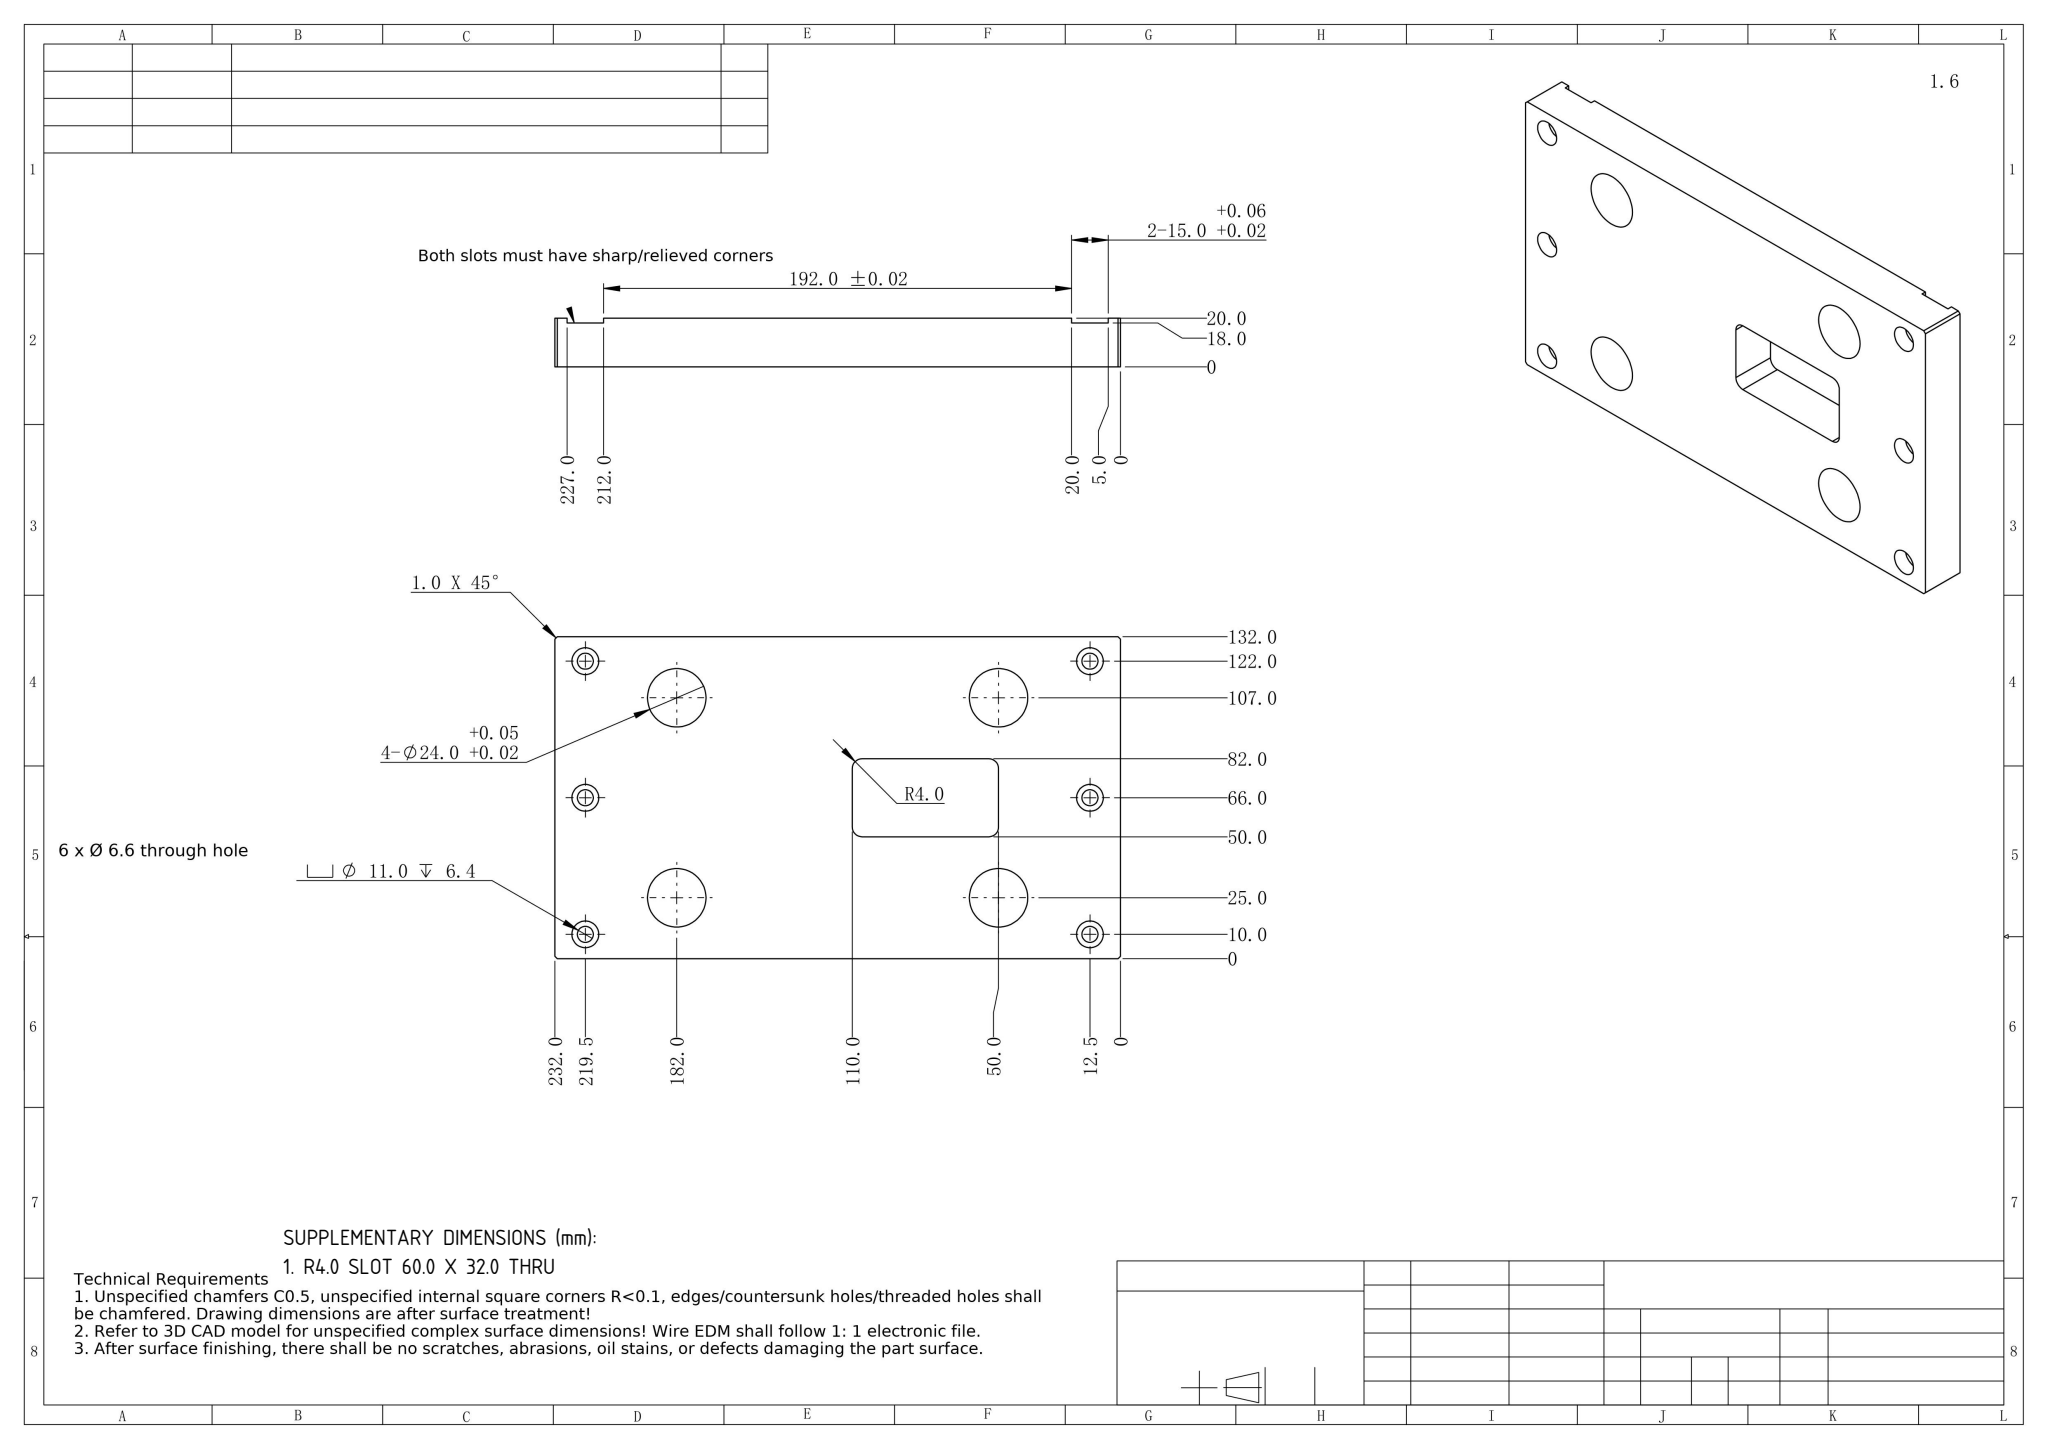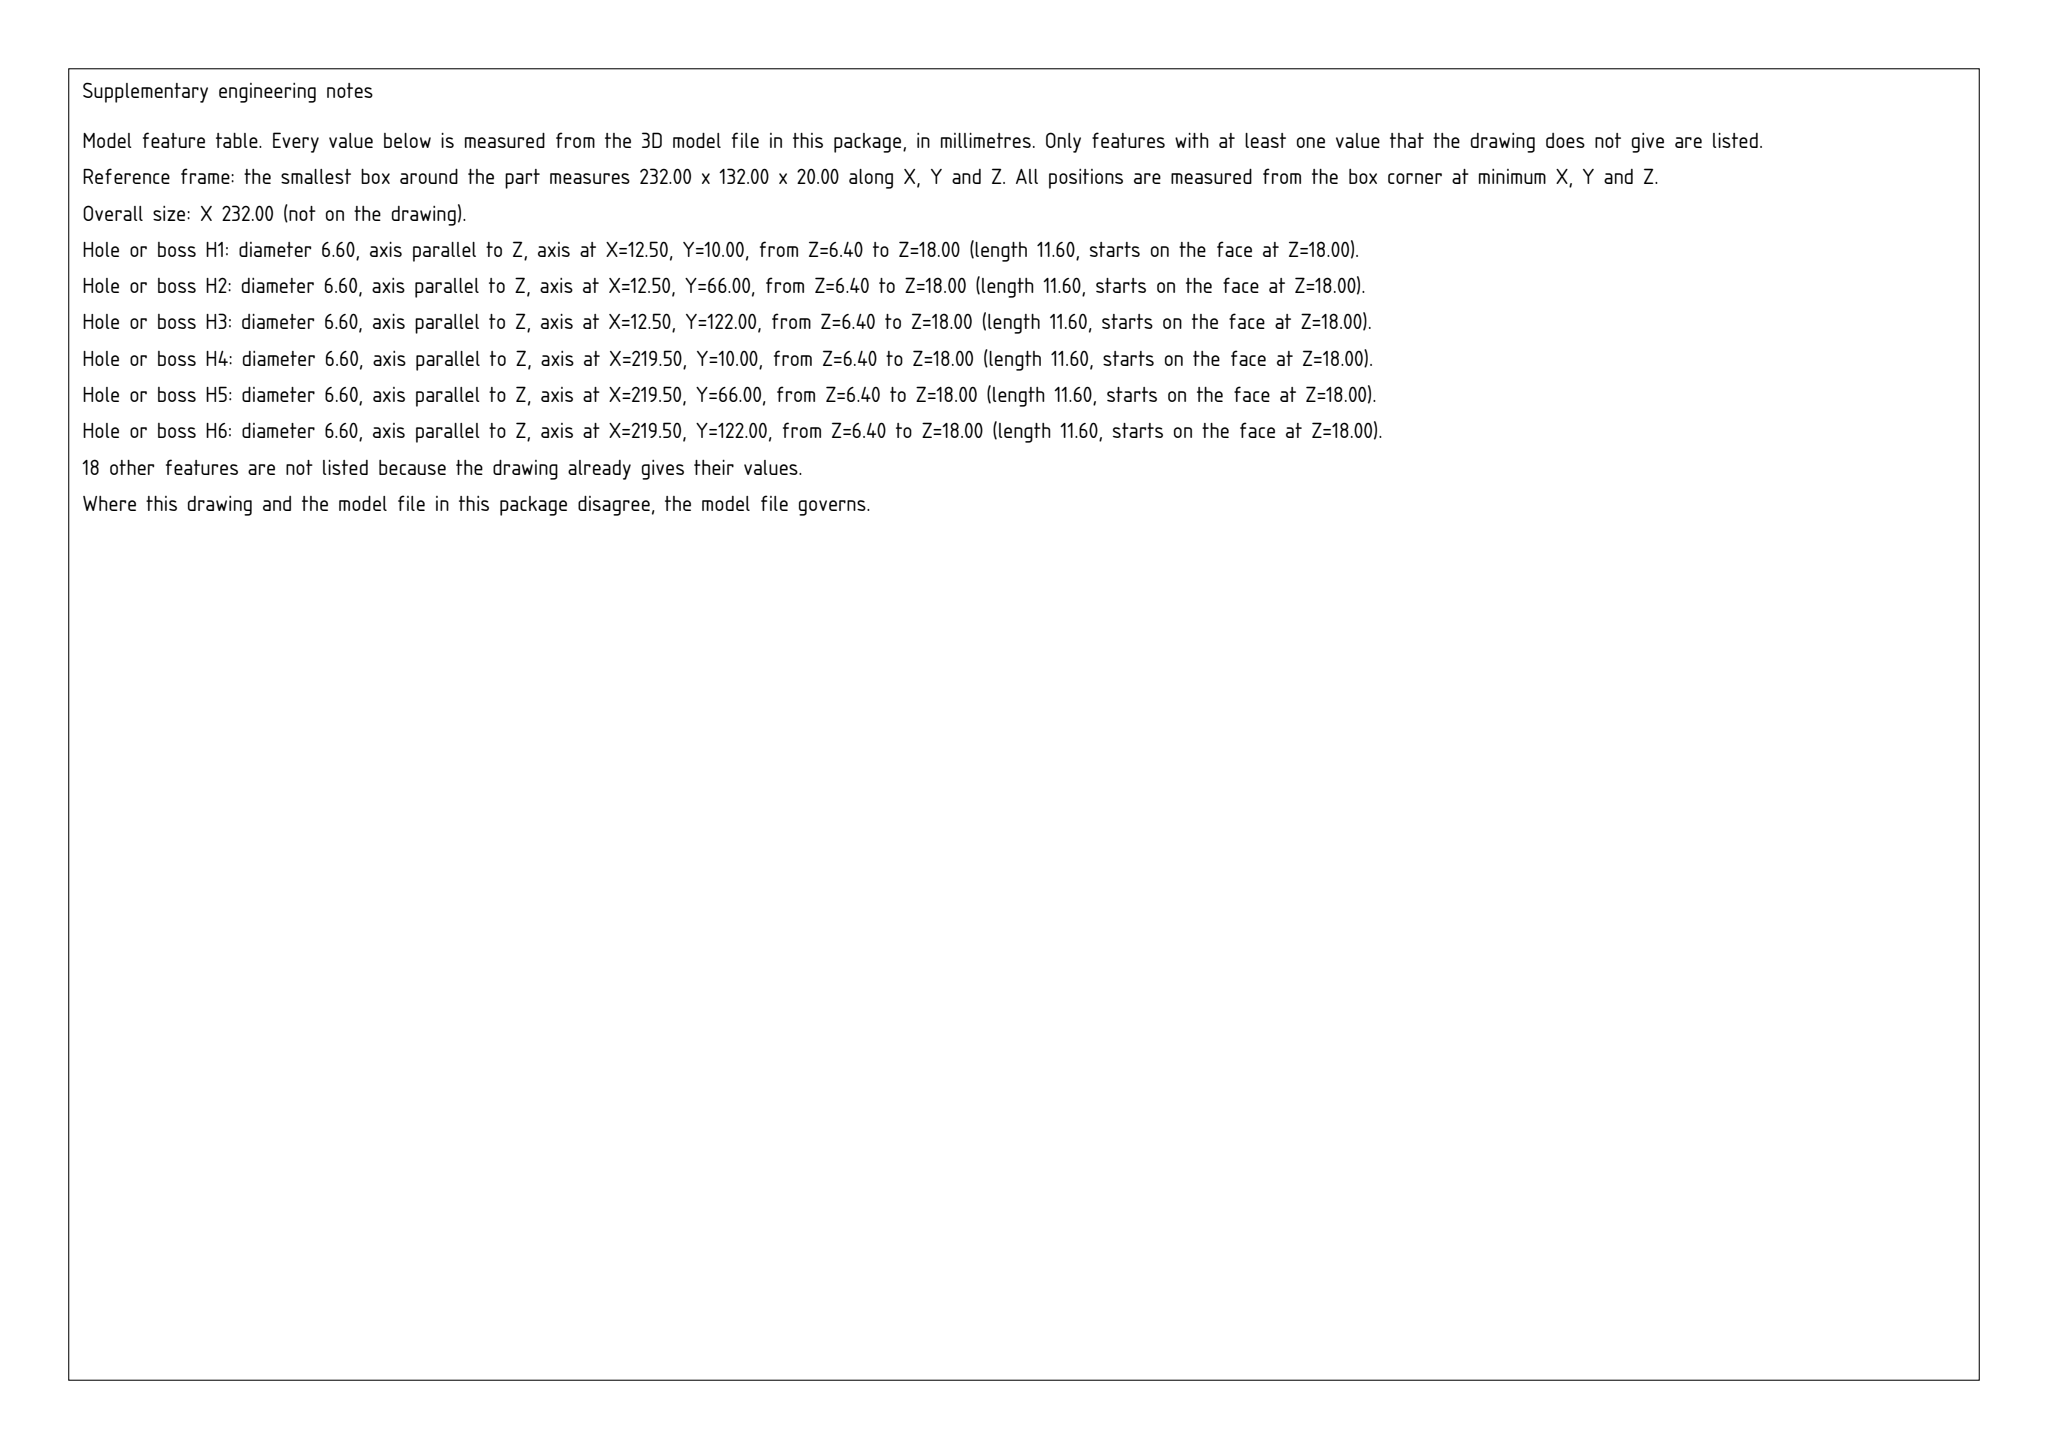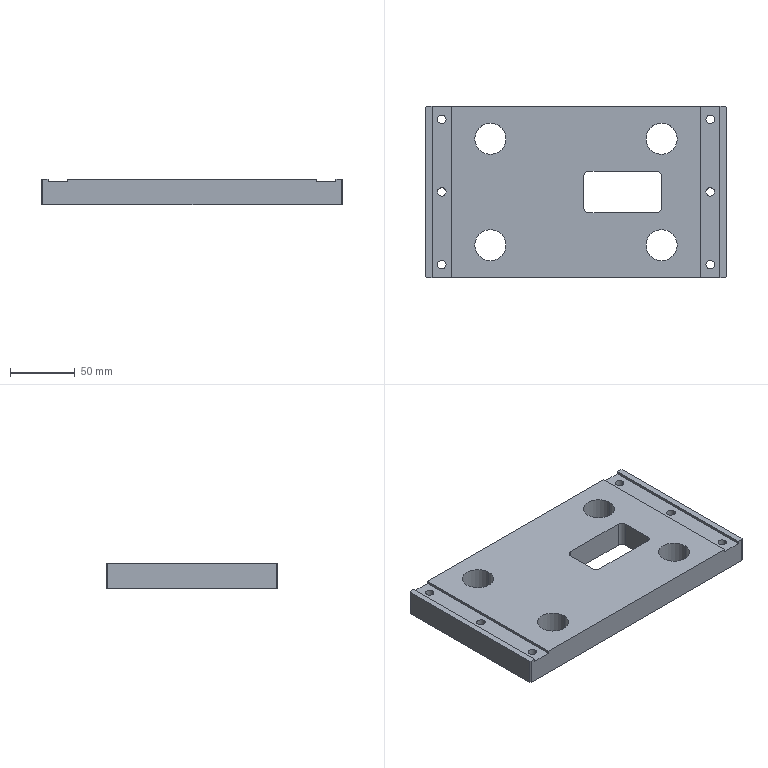Part | SolidWorks | mm | 1 solid | 64 faces | box 232 x 132 x 20 mm | volume 524173 mm3 | cylinder 36 | plane 28 | commonest cylinder face diameters 11 x12 6.6 x12 24 x8 8 x4
build123d program:
from build123d import *

# Parameters (mm, degrees)
SKETCH1_W                                       = 232
SKETCH1_H                                       = 132
BOSS_EXTRUDE1_DEPTH                             = 10
SKETCH2_W                                       = 15
SKETCH2_H                                       = 132
CUT_EXTRUDE1_DEPTH                              = 2
SKETCH3_R                                       = 12
CUT_EXTRUDE2_DEPTH                              = 268.671
SKETCH4_W                                       = 60
SKETCH4_H                                       = 32
CUT_EXTRUDE3_DEPTH                              = 268.671
FILLET1_R                                       = 4
M6_HEX_SOCKET_HEAD_CAP_SCREW_CBORE1_D           = 6.6
M6_HEX_SOCKET_HEAD_CAP_SCREW_CBORE1_CBORE_D     = 11
M6_HEX_SOCKET_HEAD_CAP_SCREW_CBORE1_CBORE_DEPTH = 6.4
CHAMFER1_SIZE                                   = 1


with BuildPart() as part:
    # Sketch1 → Boss-Extrude1 (new, symmetric)
    with BuildSketch(Plane.XY):
        with Locations((116, 66)):
            Rectangle(SKETCH1_W, SKETCH1_H)
    extrude(amount=BOSS_EXTRUDE1_DEPTH, both=True)

    # Sketch2 → Cut-Extrude1 (cut)
    with BuildSketch(Plane.XY.offset(10)):
        with Locations((12.5, 66)):
            Rectangle(SKETCH2_W, SKETCH2_H)
        with Locations((219.5, 66)):
            Rectangle(SKETCH2_W, SKETCH2_H)
    extrude(amount=-CUT_EXTRUDE1_DEPTH, mode=Mode.SUBTRACT)

    # Sketch3 → Cut-Extrude2 (cut, through all)
    with BuildSketch(Plane.XY.offset(10)):
        with Locations((50, 107)):
            Circle(SKETCH3_R)
        with Locations((182, 107)):
            Circle(SKETCH3_R)
        with Locations((50, 25)):
            Circle(SKETCH3_R)
        with Locations((182, 25)):
            Circle(SKETCH3_R)
    extrude(amount=-CUT_EXTRUDE2_DEPTH, mode=Mode.SUBTRACT)

    # Sketch4 → Cut-Extrude3 (cut, through all)
    with BuildSketch(Plane.XY.offset(10)):
        with Locations((152, 66)):
            Rectangle(SKETCH4_W, SKETCH4_H)
    extrude(amount=-CUT_EXTRUDE3_DEPTH, mode=Mode.SUBTRACT)

    # Fillet1
    fillet1_edges = [part.edges().sort_by_distance(p)[0] for p in [
        (122, 50, 0),
        (122, 82, 0),
        (182, 82, 0),
        (182, 50, 0),
    ]]
    fillet(fillet1_edges, radius=FILLET1_R)

    # M6 Hex Socket Head Cap Screw CBORE1 (through all)
    with Locations(Plane(origin=(0, 0, -10), x_dir=(-1, 0, 0), z_dir=(0, 0, -1))):
        with Locations((-12.5, 10), (-12.5, 66), (-12.5, 122), (-219.5, 10), (-219.5, 66), (-219.5, 122)):
            CounterBoreHole(M6_HEX_SOCKET_HEAD_CAP_SCREW_CBORE1_D / 2, M6_HEX_SOCKET_HEAD_CAP_SCREW_CBORE1_CBORE_D / 2, M6_HEX_SOCKET_HEAD_CAP_SCREW_CBORE1_CBORE_DEPTH)

    # Chamfer1
    chamfer1_edges = [part.edges().sort_by_distance(p)[0] for p in [
        (0, 132, 0),
        (232, 132, 0),
        (232, 0, 0),
        (0, 0, 0),
    ]]
    chamfer(chamfer1_edges, length=CHAMFER1_SIZE)


solid = part.part